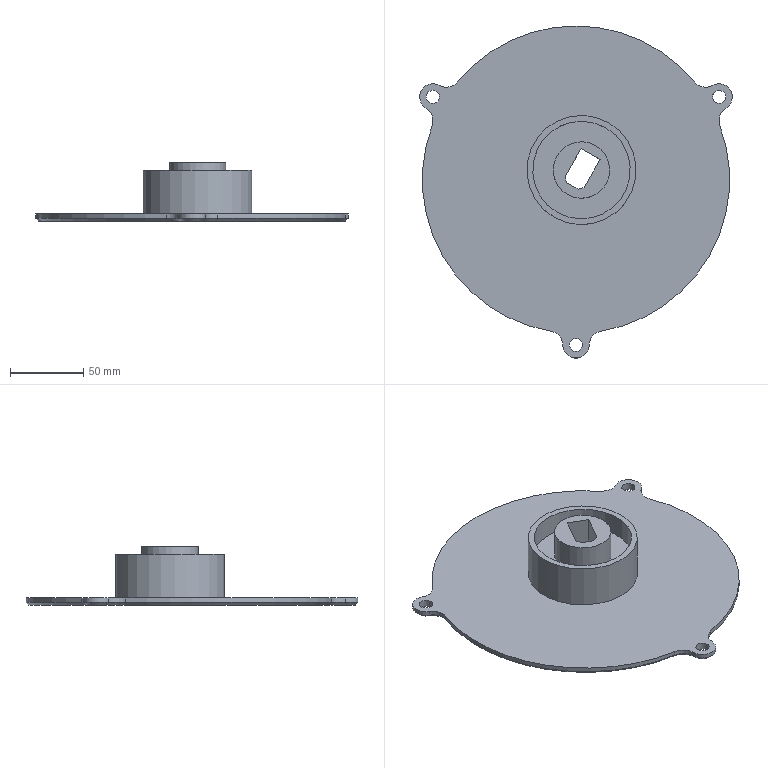Component | NX | PUMP_COVER | 1 solid | 71 faces | volume 262950 mm3 | plane 35 | cylinder 24 | cone 12 | commonest cylinder face diameters 20 x6 3 x6 210 x3 18 x3 9 x3 74.65 x1 66.65 x1 38.65 x1